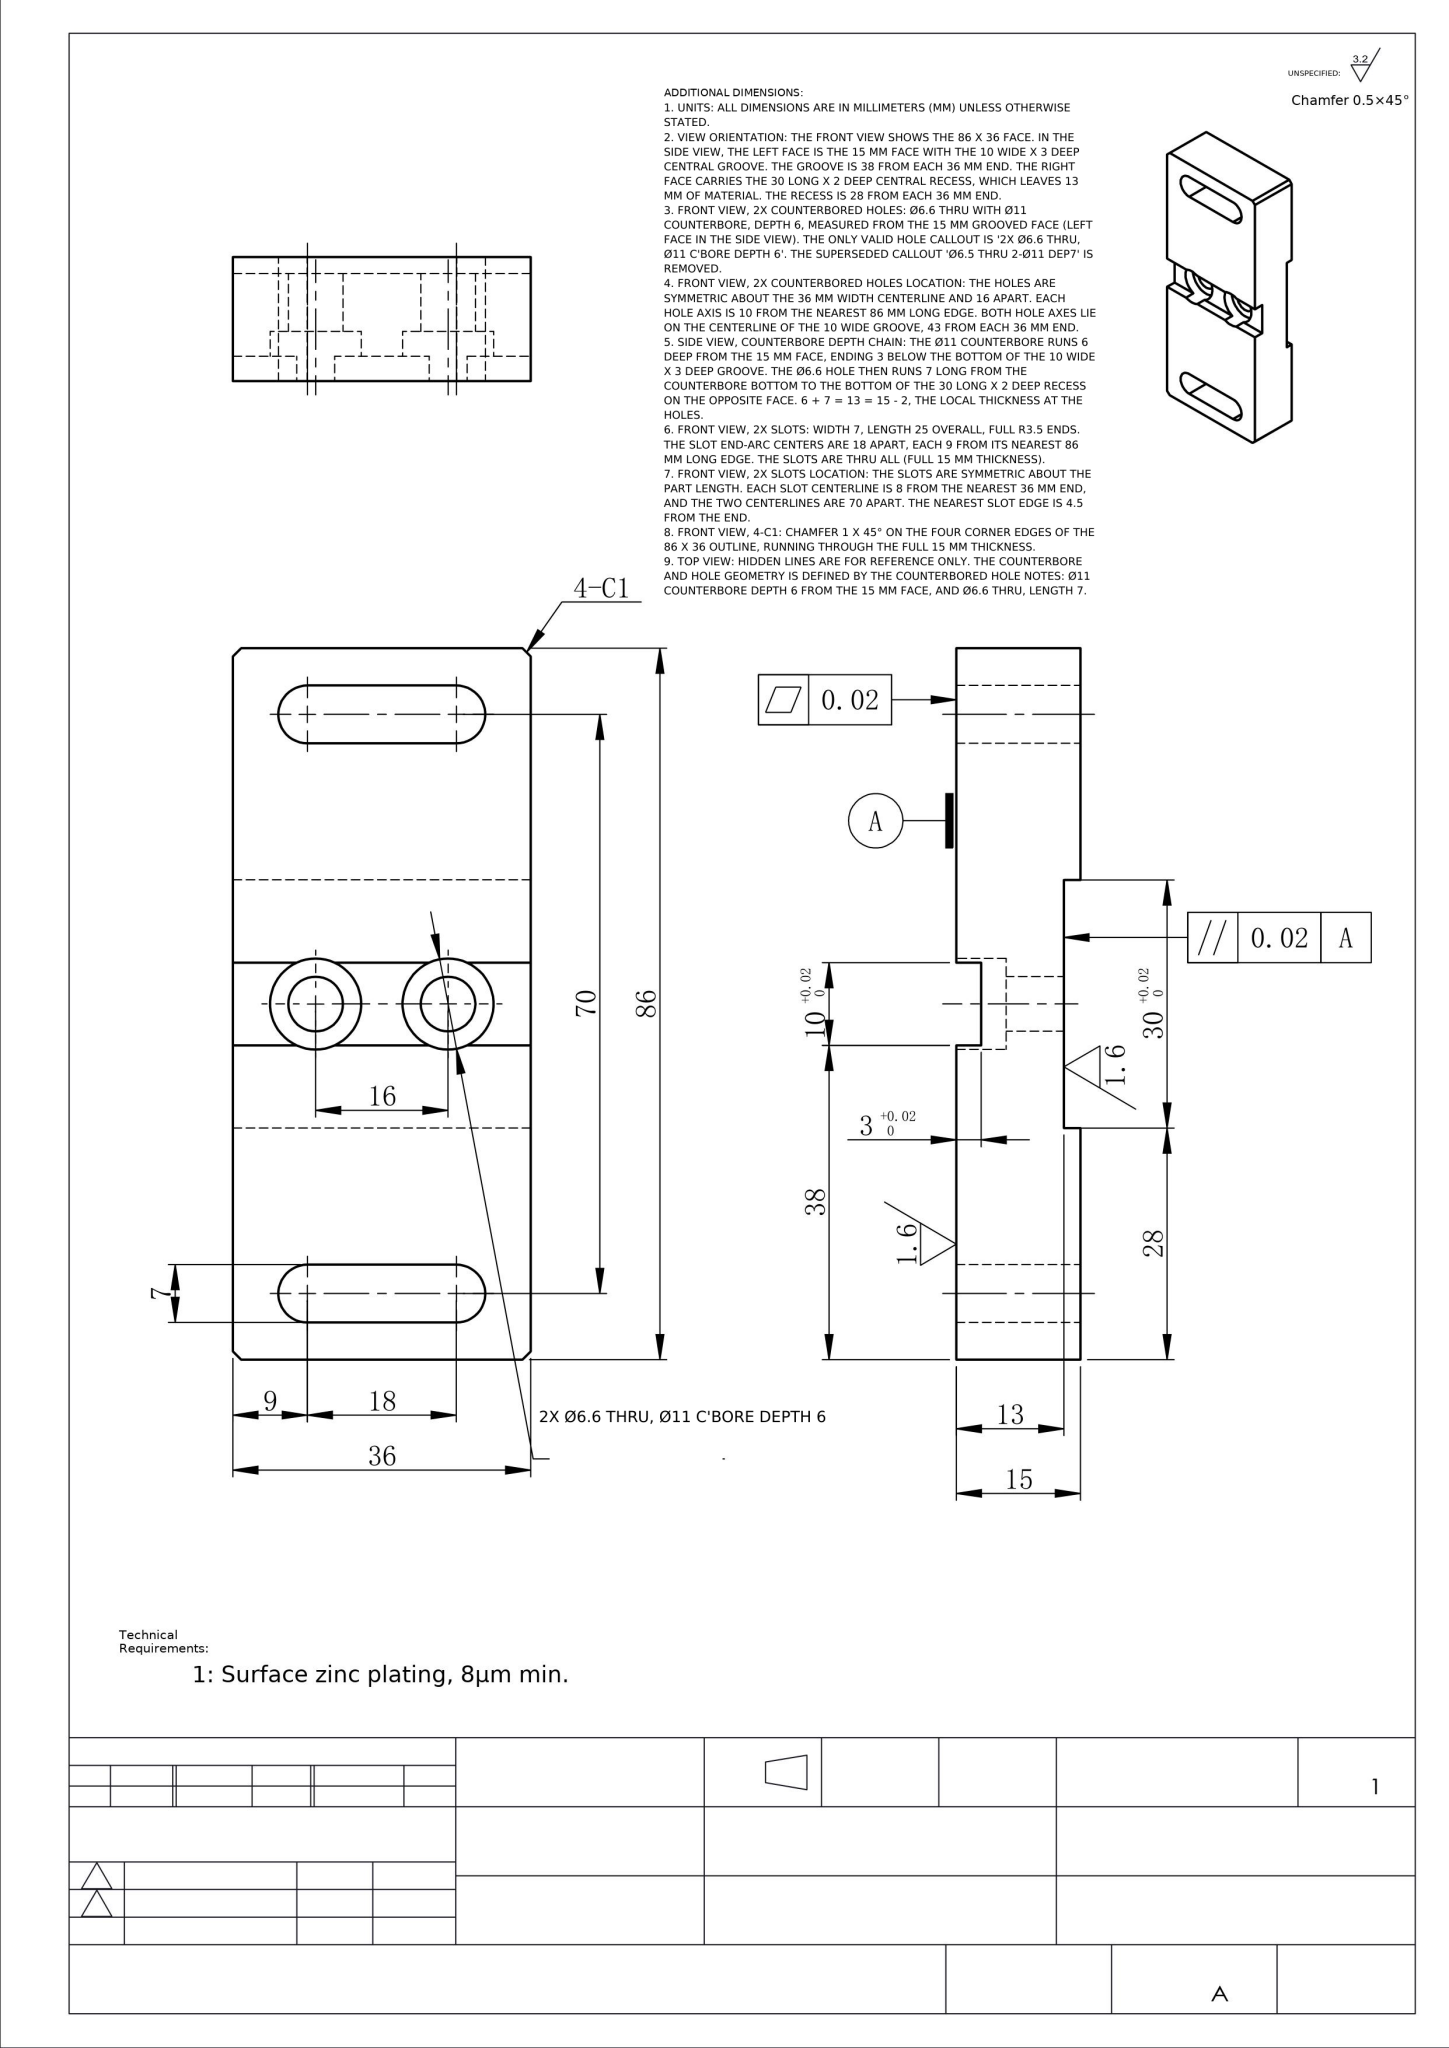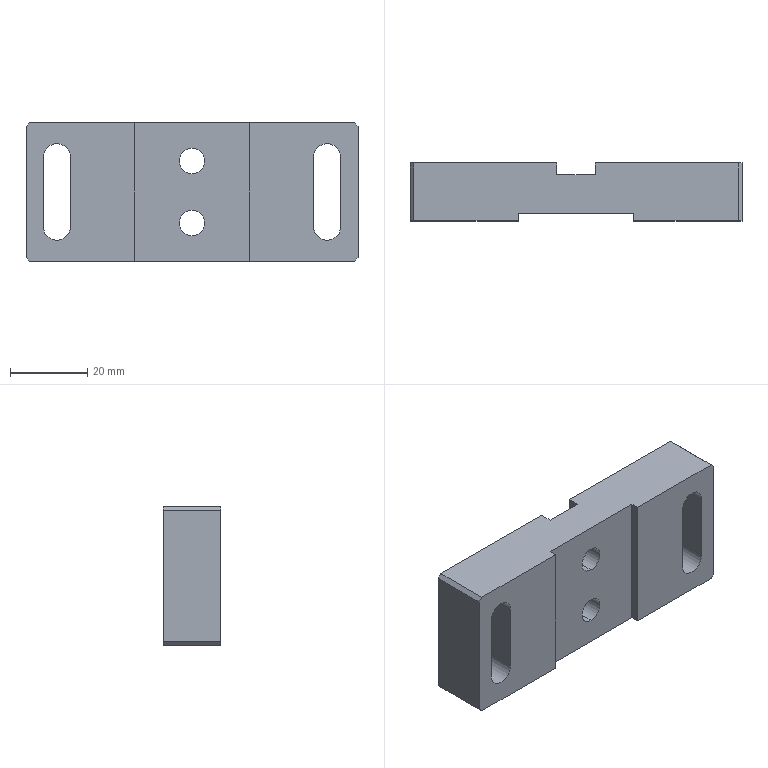Part | NX | mm | 1 solid | 44 faces | box 86 x 15 x 36 mm | volume 37168 mm3 | plane 30 | cylinder 14 | commonest cylinder face diameters 7 x6 11 x4 6.6 x4